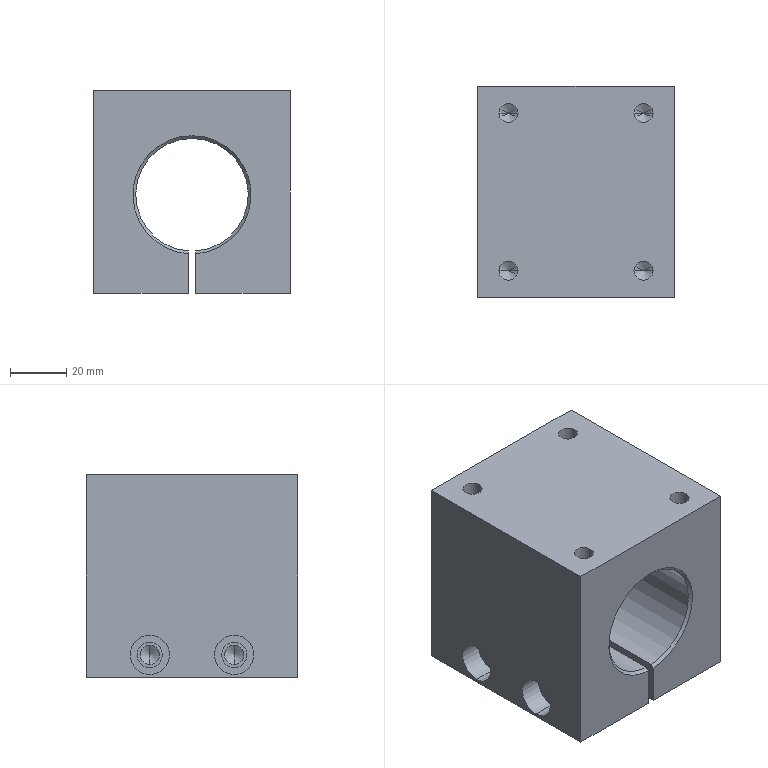Component | SolidWorks | FixedSeat-1 | 1 solid | 47 faces | box 70 x 75 x 72 mm | volume 270621 mm3 | cylinder 21 | cone 15 | plane 11 | commonest cylinder face diameters 6.8 x12 14 x4 9 x4 40 x1
build123d program:
from build123d import *

# Parameters (mm, degrees)
SKETCH1_W                                 = 70
SKETCH1_H                                 = 75
BOSS_EXTRUDE1_DEPTH                       = 36
SKETCH2_R                                 = 20
CUT_EXTRUDE1_DEPTH                        = 91.255
SKETCH3_W                                 = 2.5
SKETCH3_H                                 = 34.231
CUT_EXTRUDE2_DEPTH                        = 91.255
M8_HEX_HEAD_BOLT_COUNTERBORE1_D           = 9
M8_HEX_HEAD_BOLT_COUNTERBORE1_DEPTH       = 33
M8_HEX_HEAD_BOLT_COUNTERBORE1_CBORE_D     = 14
M8_HEX_HEAD_BOLT_COUNTERBORE1_CBORE_DEPTH = 8
M8_HEX_HEAD_BOLT_COUNTERBORE1_TIP         = 2.704
CUT_EXTRUDE3_START                        = -25.75
SKETCH6_R                                 = 4.5
CUT_EXTRUDE3_DEPTH                        = 25.75
M8_TAPPED_HOLE1_D                         = 6.8
M8_TAPPED_HOLE1_DEPTH                     = 19.75
M8_TAPPED_HOLE1_TIP                       = 2.043
M8_TAPPED_HOLE2_D                         = 6.8
M8_TAPPED_HOLE2_DEPTH                     = 19.75
M8_TAPPED_HOLE2_TIP                       = 2.043
CHAMFER1_SIZE                             = 1


with BuildPart() as part:
    # Sketch1 → Boss-Extrude1 (new, symmetric)
    with BuildSketch(Plane.XY):
        Rectangle(SKETCH1_W, SKETCH1_H)
    extrude(amount=BOSS_EXTRUDE1_DEPTH, both=True)

    # Sketch2 → Cut-Extrude1 (cut, through all)
    with BuildSketch(Plane(origin=(0, 37.5, 0), x_dir=(1, 0, 0), z_dir=(0, 1, 0))):
        with Locations(Location((0, -1, 0), (0, 0, 270))):
            Circle(SKETCH2_R)
    extrude(amount=-CUT_EXTRUDE1_DEPTH, mode=Mode.SUBTRACT)

    # Sketch3 → Cut-Extrude2 (cut, through all)
    with BuildSketch(Plane(origin=(0, 37.5, 0), x_dir=(1, 0, 0), z_dir=(0, 1, 0))):
        with Locations((0, -25.561)):
            Rectangle(SKETCH3_W, SKETCH3_H)
    extrude(amount=-CUT_EXTRUDE2_DEPTH, mode=Mode.SUBTRACT)

    # M8 Hex Head Bolt Counterbore1
    with Locations(Plane(origin=(35, 0, 0), x_dir=(0, 0, -1), z_dir=(1, 0, 0))):
        with Locations((-28, 15), (-28, -15)):
            CounterBoreHole(M8_HEX_HEAD_BOLT_COUNTERBORE1_D / 2, M8_HEX_HEAD_BOLT_COUNTERBORE1_CBORE_D / 2, M8_HEX_HEAD_BOLT_COUNTERBORE1_CBORE_DEPTH, depth=M8_HEX_HEAD_BOLT_COUNTERBORE1_DEPTH)
            with Locations((0, 0, -(M8_HEX_HEAD_BOLT_COUNTERBORE1_DEPTH + M8_HEX_HEAD_BOLT_COUNTERBORE1_TIP / 2))):  # 118° drill point
                Cone(0, M8_HEX_HEAD_BOLT_COUNTERBORE1_D / 2, M8_HEX_HEAD_BOLT_COUNTERBORE1_TIP, mode=Mode.SUBTRACT)

    # Sketch6 → Cut-Extrude3 (cut)
    with BuildSketch(Plane(origin=(27, 0, 0), x_dir=(0, 0, -1), z_dir=(1, 0, 0)).offset(CUT_EXTRUDE3_START)):
        with Locations((-28, 15)):
            Circle(SKETCH6_R)
        with Locations((-28, -15)):
            Circle(SKETCH6_R)
    extrude(amount=CUT_EXTRUDE3_DEPTH, mode=Mode.SUBTRACT)

    # M8 Tapped Hole1
    with Locations(Plane(origin=(-1.25, 0, 0), x_dir=(0, 0, -1), z_dir=(1, 0, 0))):
        with Locations((-28, 15), (-28, -15)):
            Hole(M8_TAPPED_HOLE1_D / 2, depth=M8_TAPPED_HOLE1_DEPTH)
            with Locations((0, 0, -(M8_TAPPED_HOLE1_DEPTH + M8_TAPPED_HOLE1_TIP / 2))):  # 118° drill point
                Cone(0, M8_TAPPED_HOLE1_D / 2, M8_TAPPED_HOLE1_TIP, mode=Mode.SUBTRACT)

    # M8 Tapped Hole2
    with Locations(Plane(origin=(0, 0, -36), x_dir=(-1, 0, 0), z_dir=(0, 0, -1))):
        with Locations((-24, 28), (-24, -28), (24, 28), (24, -28)):
            Hole(M8_TAPPED_HOLE2_D / 2, depth=M8_TAPPED_HOLE2_DEPTH)
            with Locations((0, 0, -(M8_TAPPED_HOLE2_DEPTH + M8_TAPPED_HOLE2_TIP / 2))):  # 118° drill point
                Cone(0, M8_TAPPED_HOLE2_D / 2, M8_TAPPED_HOLE2_TIP, mode=Mode.SUBTRACT)

    # Chamfer1
    chamfer1_edges = [part.edges().sort_by_distance(p)[0] for p in [
        (0, -37.5, -19),
        (0, 37.5, -19),
    ]]
    chamfer(chamfer1_edges, length=CHAMFER1_SIZE)


solid = part.part

# Placed as in the assembly
solid = solid.moved(Location((-194.507, -206.911, 459), (-180, 0, 180)))